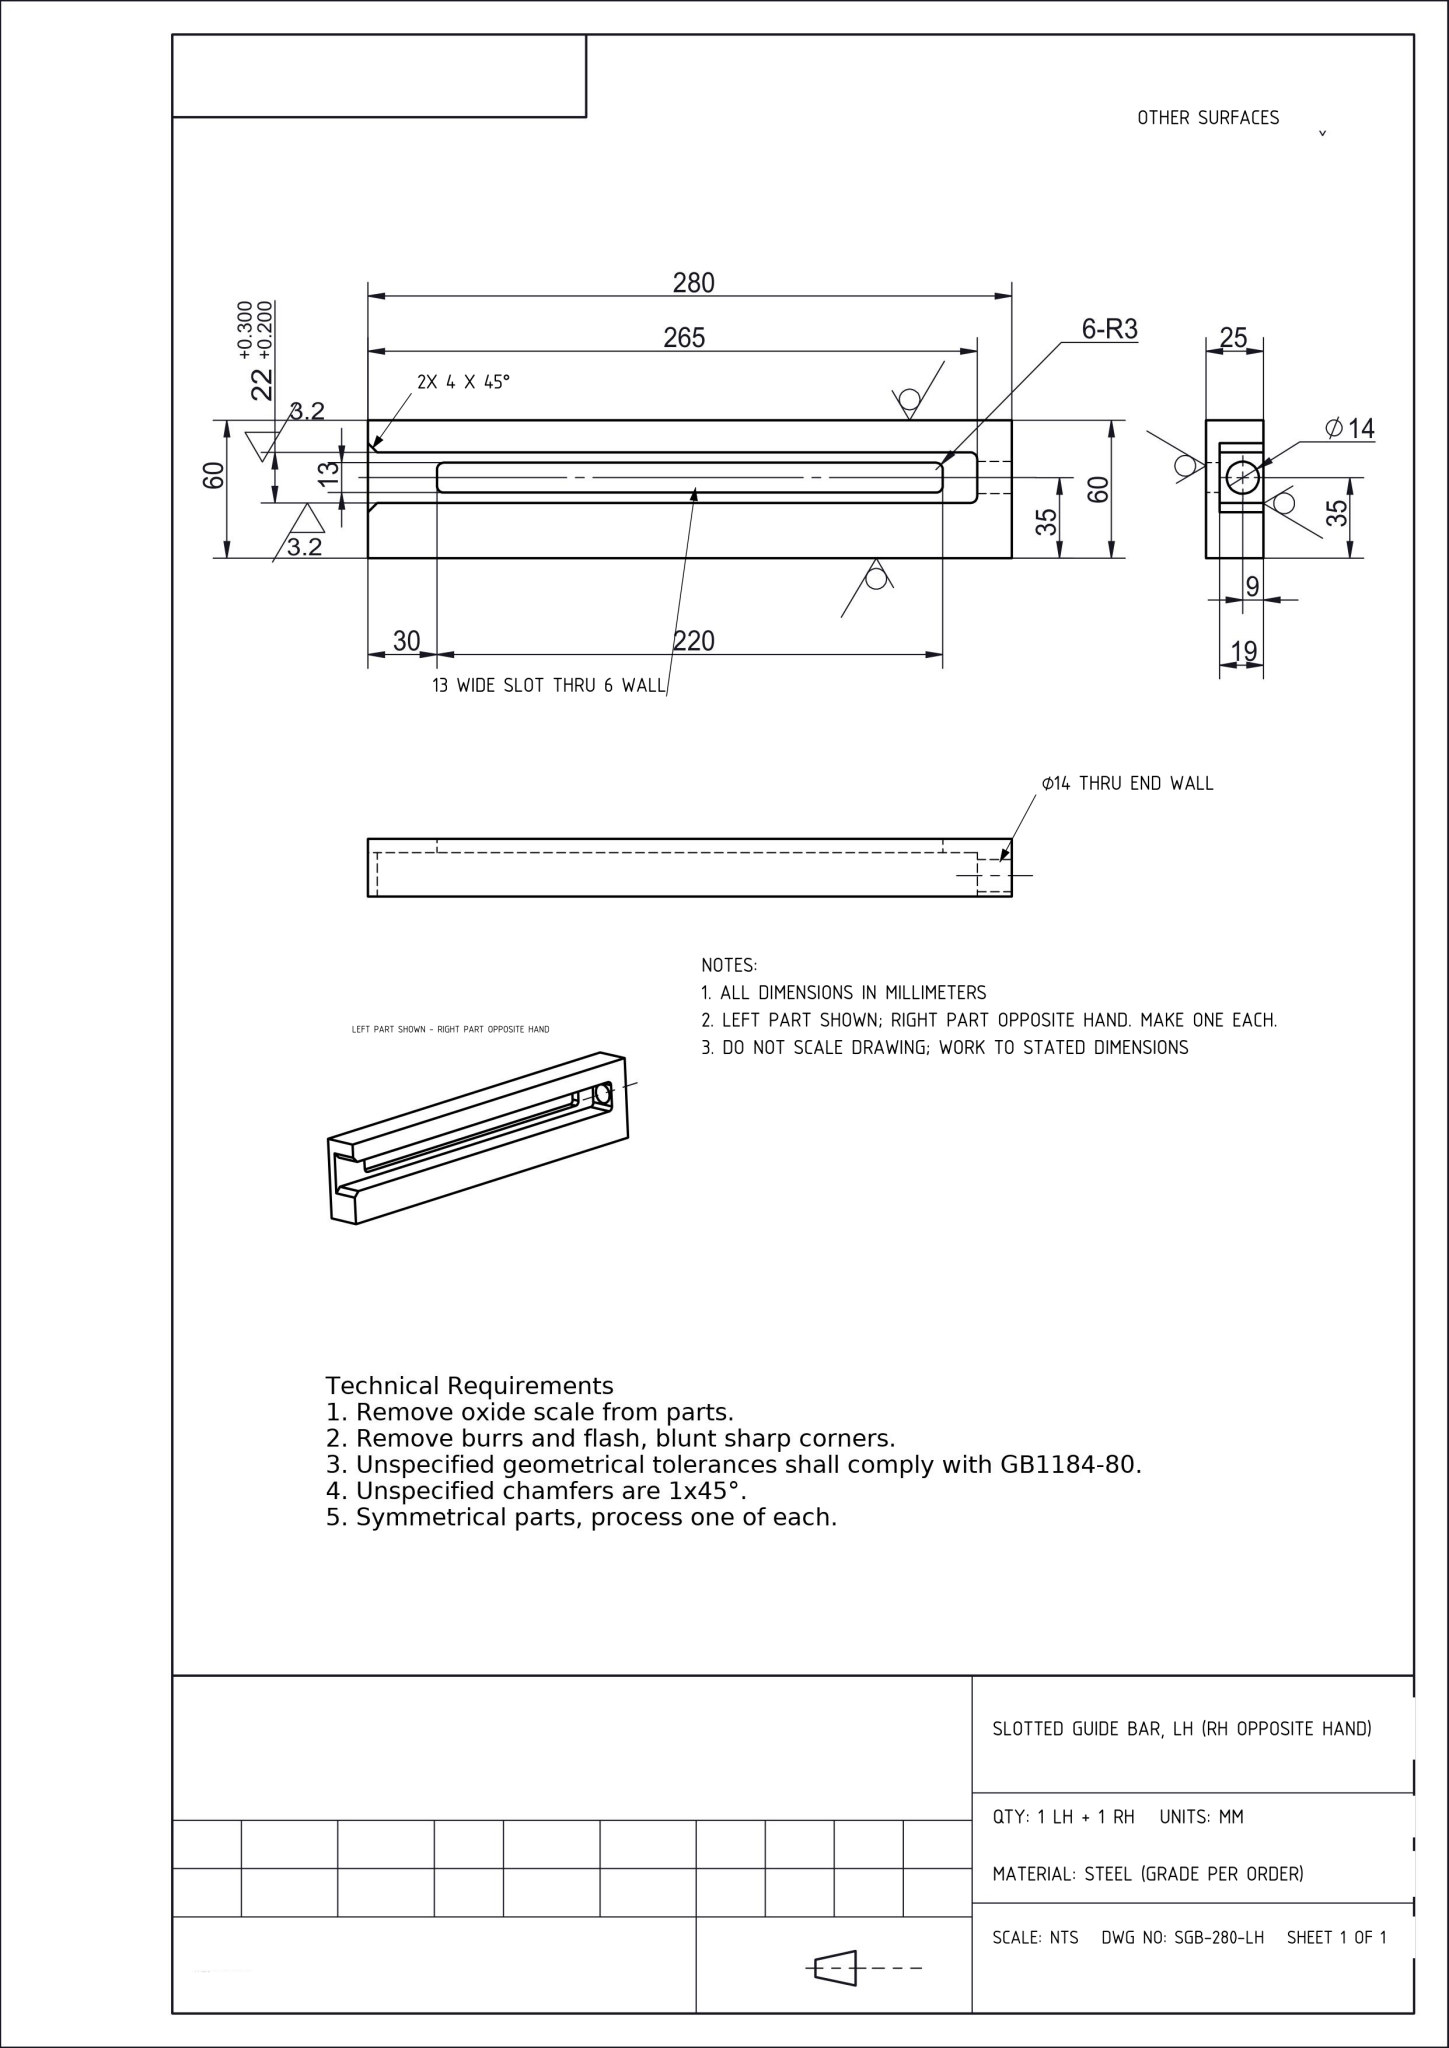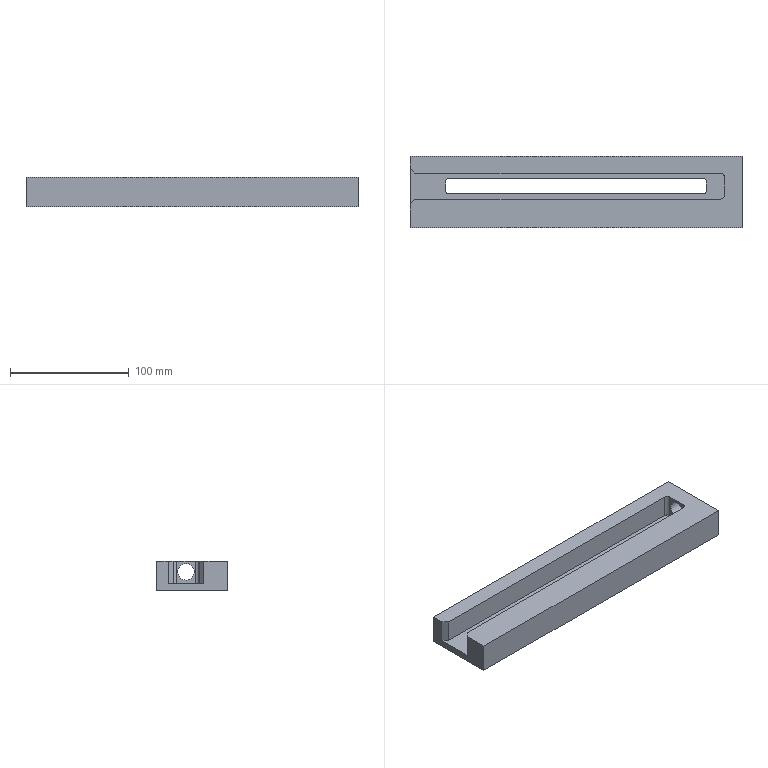Part | NX | mm | 1 solid | 24 faces | box 280 x 60 x 25 mm | volume 289577 mm3 | plane 16 | cylinder 8 | commonest cylinder face diameters 6 x6 14 x2
STEP:
#1=COLOUR_RGB('',1.,1.,1.);
#2=FILL_AREA_STYLE_COLOUR('',#1);
#3=FILL_AREA_STYLE('',(#2));
#4=SURFACE_STYLE_FILL_AREA(#3);
#5=SURFACE_SIDE_STYLE('',(#4));
#6=SURFACE_STYLE_USAGE(.BOTH.,#5);
#7=PRESENTATION_STYLE_ASSIGNMENT((#6));
#8=CARTESIAN_POINT('',(125.,5.,23.));
#9=VERTEX_POINT('',#8);
#10=CARTESIAN_POINT('',(125.,5.,9.));
#11=VERTEX_POINT('',#10);
#12=CARTESIAN_POINT('',(125.,5.,16.));
#13=DIRECTION('',(1.,-0.,-0.));
#14=DIRECTION('',(0.,0.,-1.));
#15=AXIS2_PLACEMENT_3D('',#12,#13,#14);
#16=CIRCLE('',#15,7.);
#17=EDGE_CURVE('',#9,#11,#16,.T.);
#18=ORIENTED_EDGE('',*,*,#17,.F.);
#19=CARTESIAN_POINT('',(140.,5.,23.));
#20=VERTEX_POINT('',#19);
#21=CARTESIAN_POINT('',(140.,5.,23.));
#22=DIRECTION('',(1.,-0.,-0.));
#23=VECTOR('',#22,1000.);
#24=LINE('',#21,#23);
#25=EDGE_CURVE('',#9,#20,#24,.T.);
#26=ORIENTED_EDGE('',*,*,#25,.T.);
#27=CARTESIAN_POINT('',(140.,5.,9.));
#28=VERTEX_POINT('',#27);
#29=CARTESIAN_POINT('',(140.,5.,16.));
#30=DIRECTION('',(1.,-0.,-0.));
#31=DIRECTION('',(0.,0.,-1.));
#32=AXIS2_PLACEMENT_3D('',#29,#30,#31);
#33=CIRCLE('',#32,7.);
#34=EDGE_CURVE('',#20,#28,#33,.T.);
#35=ORIENTED_EDGE('',*,*,#34,.T.);
#36=CARTESIAN_POINT('',(140.,5.,9.));
#37=DIRECTION('',(1.,-0.,-0.));
#38=VECTOR('',#37,1000.);
#39=LINE('',#36,#38);
#40=EDGE_CURVE('',#11,#28,#39,.T.);
#41=ORIENTED_EDGE('',*,*,#40,.F.);
#42=EDGE_LOOP('',(#18,#26,#35,#41));
#43=FACE_OUTER_BOUND('',#42,.T.);
#44=CARTESIAN_POINT('',(140.,5.,16.));
#45=DIRECTION('',(1.,-0.,-0.));
#46=DIRECTION('',(0.,0.,-1.));
#47=AXIS2_PLACEMENT_3D('',#44,#45,#46);
#48=CYLINDRICAL_SURFACE('',#47,7.);
#49=ADVANCED_FACE('',(#43),#48,.F.);
#50=CARTESIAN_POINT('',(140.,5.,16.));
#51=DIRECTION('',(1.,-0.,-0.));
#52=DIRECTION('',(0.,0.,-1.));
#53=AXIS2_PLACEMENT_3D('',#50,#51,#52);
#54=CIRCLE('',#53,7.);
#55=EDGE_CURVE('',#28,#20,#54,.T.);
#56=ORIENTED_EDGE('',*,*,#55,.F.);
#57=ORIENTED_EDGE('',*,*,#34,.F.);
#58=EDGE_LOOP('',(#56,#57));
#59=FACE_BOUND('',#58,.T.);
#60=CARTESIAN_POINT('',(140.,-30.,0.));
#61=VERTEX_POINT('',#60);
#62=CARTESIAN_POINT('',(140.,30.,0.));
#63=VERTEX_POINT('',#62);
#64=CARTESIAN_POINT('',(140.,30.,0.));
#65=DIRECTION('',(-0.,1.,-0.));
#66=VECTOR('',#65,1000.);
#67=LINE('',#64,#66);
#68=EDGE_CURVE('',#61,#63,#67,.T.);
#69=ORIENTED_EDGE('',*,*,#68,.T.);
#70=CARTESIAN_POINT('',(140.,30.,25.));
#71=VERTEX_POINT('',#70);
#72=CARTESIAN_POINT('',(140.,30.,25.));
#73=DIRECTION('',(0.,0.,-1.));
#74=VECTOR('',#73,1000.);
#75=LINE('',#72,#74);
#76=EDGE_CURVE('',#71,#63,#75,.T.);
#77=ORIENTED_EDGE('',*,*,#76,.F.);
#78=CARTESIAN_POINT('',(140.,-30.,25.));
#79=VERTEX_POINT('',#78);
#80=CARTESIAN_POINT('',(140.,30.,25.));
#81=DIRECTION('',(-0.,1.,-0.));
#82=VECTOR('',#81,1000.);
#83=LINE('',#80,#82);
#84=EDGE_CURVE('',#79,#71,#83,.T.);
#85=ORIENTED_EDGE('',*,*,#84,.F.);
#86=CARTESIAN_POINT('',(140.,-30.,25.));
#87=DIRECTION('',(0.,0.,-1.));
#88=VECTOR('',#87,1000.);
#89=LINE('',#86,#88);
#90=EDGE_CURVE('',#79,#61,#89,.T.);
#91=ORIENTED_EDGE('',*,*,#90,.T.);
#92=EDGE_LOOP('',(#69,#77,#85,#91));
#93=FACE_OUTER_BOUND('',#92,.T.);
#94=CARTESIAN_POINT('',(140.,30.,25.));
#95=DIRECTION('',(-1.,0.,-0.));
#96=DIRECTION('',(-0.,-0.,1.));
#97=AXIS2_PLACEMENT_3D('',#94,#95,#96);
#98=PLANE('',#97);
#99=ADVANCED_FACE('',(#59,#93),#98,.F.);
#100=CARTESIAN_POINT('',(-140.,30.,0.));
#101=VERTEX_POINT('',#100);
#102=CARTESIAN_POINT('',(-140.,30.,0.));
#103=DIRECTION('',(-1.,0.,0.));
#104=VECTOR('',#103,1000.);
#105=LINE('',#102,#104);
#106=EDGE_CURVE('',#63,#101,#105,.T.);
#107=ORIENTED_EDGE('',*,*,#106,.T.);
#108=CARTESIAN_POINT('',(-140.,30.,25.));
#109=VERTEX_POINT('',#108);
#110=CARTESIAN_POINT('',(-140.,30.,25.));
#111=DIRECTION('',(0.,0.,-1.));
#112=VECTOR('',#111,1000.);
#113=LINE('',#110,#112);
#114=EDGE_CURVE('',#109,#101,#113,.T.);
#115=ORIENTED_EDGE('',*,*,#114,.F.);
#116=CARTESIAN_POINT('',(-140.,30.,25.));
#117=DIRECTION('',(-1.,0.,0.));
#118=VECTOR('',#117,1000.);
#119=LINE('',#116,#118);
#120=EDGE_CURVE('',#71,#109,#119,.T.);
#121=ORIENTED_EDGE('',*,*,#120,.F.);
#122=ORIENTED_EDGE('',*,*,#76,.T.);
#123=EDGE_LOOP('',(#107,#115,#121,#122));
#124=FACE_OUTER_BOUND('',#123,.T.);
#125=CARTESIAN_POINT('',(-140.,30.,25.));
#126=DIRECTION('',(0.,-1.,-0.));
#127=DIRECTION('',(0.,0.,-1.));
#128=AXIS2_PLACEMENT_3D('',#125,#126,#127);
#129=PLANE('',#128);
#130=ADVANCED_FACE('',(#124),#129,.F.);
#131=CARTESIAN_POINT('',(-140.,-10.,25.));
#132=VERTEX_POINT('',#131);
#133=CARTESIAN_POINT('',(-140.,-30.,25.));
#134=VERTEX_POINT('',#133);
#135=CARTESIAN_POINT('',(-140.,30.,25.));
#136=DIRECTION('',(0.,-1.,0.));
#137=VECTOR('',#136,1000.);
#138=LINE('',#135,#137);
#139=EDGE_CURVE('',#132,#134,#138,.T.);
#140=ORIENTED_EDGE('',*,*,#139,.F.);
#141=CARTESIAN_POINT('',(-140.,-10.,6.));
#142=VERTEX_POINT('',#141);
#143=CARTESIAN_POINT('',(-140.,-10.,25.));
#144=DIRECTION('',(-0.,-0.,-1.));
#145=VECTOR('',#144,1000.);
#146=LINE('',#143,#145);
#147=EDGE_CURVE('',#132,#142,#146,.T.);
#148=ORIENTED_EDGE('',*,*,#147,.T.);
#149=CARTESIAN_POINT('',(-140.,20.,6.));
#150=VERTEX_POINT('',#149);
#151=CARTESIAN_POINT('',(-140.,30.,6.));
#152=DIRECTION('',(0.,-1.,0.));
#153=VECTOR('',#152,1000.);
#154=LINE('',#151,#153);
#155=EDGE_CURVE('',#150,#142,#154,.T.);
#156=ORIENTED_EDGE('',*,*,#155,.F.);
#157=CARTESIAN_POINT('',(-140.,20.,25.));
#158=VERTEX_POINT('',#157);
#159=CARTESIAN_POINT('',(-140.,20.,25.));
#160=DIRECTION('',(0.,0.,1.));
#161=VECTOR('',#160,1000.);
#162=LINE('',#159,#161);
#163=EDGE_CURVE('',#150,#158,#162,.T.);
#164=ORIENTED_EDGE('',*,*,#163,.T.);
#165=CARTESIAN_POINT('',(-140.,30.,25.));
#166=DIRECTION('',(0.,-1.,0.));
#167=VECTOR('',#166,1000.);
#168=LINE('',#165,#167);
#169=EDGE_CURVE('',#109,#158,#168,.T.);
#170=ORIENTED_EDGE('',*,*,#169,.F.);
#171=ORIENTED_EDGE('',*,*,#114,.T.);
#172=CARTESIAN_POINT('',(-140.,-30.,0.));
#173=VERTEX_POINT('',#172);
#174=CARTESIAN_POINT('',(-140.,30.,0.));
#175=DIRECTION('',(0.,-1.,0.));
#176=VECTOR('',#175,1000.);
#177=LINE('',#174,#176);
#178=EDGE_CURVE('',#101,#173,#177,.T.);
#179=ORIENTED_EDGE('',*,*,#178,.T.);
#180=CARTESIAN_POINT('',(-140.,-30.,25.));
#181=DIRECTION('',(0.,0.,-1.));
#182=VECTOR('',#181,1000.);
#183=LINE('',#180,#182);
#184=EDGE_CURVE('',#134,#173,#183,.T.);
#185=ORIENTED_EDGE('',*,*,#184,.F.);
#186=EDGE_LOOP('',(#140,#148,#156,#164,#170,#171,#179,#185));
#187=FACE_OUTER_BOUND('',#186,.T.);
#188=CARTESIAN_POINT('',(-140.,30.,25.));
#189=DIRECTION('',(1.,-0.,0.));
#190=DIRECTION('',(0.,0.,-1.));
#191=AXIS2_PLACEMENT_3D('',#188,#189,#190);
#192=PLANE('',#191);
#193=ADVANCED_FACE('',(#187),#192,.F.);
#194=CARTESIAN_POINT('',(-140.,-30.,0.));
#195=DIRECTION('',(1.,-0.,-0.));
#196=VECTOR('',#195,1000.);
#197=LINE('',#194,#196);
#198=EDGE_CURVE('',#173,#61,#197,.T.);
#199=ORIENTED_EDGE('',*,*,#198,.T.);
#200=ORIENTED_EDGE('',*,*,#90,.F.);
#201=CARTESIAN_POINT('',(-140.,-30.,25.));
#202=DIRECTION('',(1.,-0.,-0.));
#203=VECTOR('',#202,1000.);
#204=LINE('',#201,#203);
#205=EDGE_CURVE('',#134,#79,#204,.T.);
#206=ORIENTED_EDGE('',*,*,#205,.F.);
#207=ORIENTED_EDGE('',*,*,#184,.T.);
#208=EDGE_LOOP('',(#199,#200,#206,#207));
#209=FACE_OUTER_BOUND('',#208,.T.);
#210=CARTESIAN_POINT('',(-140.,-30.,25.));
#211=DIRECTION('',(-0.,1.,0.));
#212=DIRECTION('',(-0.,-0.,1.));
#213=AXIS2_PLACEMENT_3D('',#210,#211,#212);
#214=PLANE('',#213);
#215=ADVANCED_FACE('',(#209),#214,.F.);
#216=CARTESIAN_POINT('',(-136.,-6.,25.));
#217=VERTEX_POINT('',#216);
#218=CARTESIAN_POINT('',(122.,-6.,25.));
#219=VERTEX_POINT('',#218);
#220=CARTESIAN_POINT('',(0.,-6.,25.));
#221=DIRECTION('',(1.,0.,-0.));
#222=VECTOR('',#221,1000.);
#223=LINE('',#220,#222);
#224=EDGE_CURVE('',#217,#219,#223,.T.);
#225=ORIENTED_EDGE('',*,*,#224,.F.);
#226=CARTESIAN_POINT('',(-65.,65.,25.));
#227=DIRECTION('',(-0.7071,-0.7071,-0.));
#228=VECTOR('',#227,1000.);
#229=LINE('',#226,#228);
#230=EDGE_CURVE('',#217,#132,#229,.T.);
#231=ORIENTED_EDGE('',*,*,#230,.T.);
#232=ORIENTED_EDGE('',*,*,#139,.T.);
#233=ORIENTED_EDGE('',*,*,#205,.T.);
#234=ORIENTED_EDGE('',*,*,#84,.T.);
#235=ORIENTED_EDGE('',*,*,#120,.T.);
#236=ORIENTED_EDGE('',*,*,#169,.T.);
#237=CARTESIAN_POINT('',(-136.,16.,25.));
#238=VERTEX_POINT('',#237);
#239=CARTESIAN_POINT('',(-60.,-60.,25.));
#240=DIRECTION('',(0.7071,-0.7071,-0.));
#241=VECTOR('',#240,1000.);
#242=LINE('',#239,#241);
#243=EDGE_CURVE('',#158,#238,#242,.T.);
#244=ORIENTED_EDGE('',*,*,#243,.T.);
#245=CARTESIAN_POINT('',(122.,16.,25.));
#246=VERTEX_POINT('',#245);
#247=CARTESIAN_POINT('',(-284.054,16.,25.));
#248=DIRECTION('',(-1.,0.,0.));
#249=VECTOR('',#248,1000.);
#250=LINE('',#247,#249);
#251=EDGE_CURVE('',#246,#238,#250,.T.);
#252=ORIENTED_EDGE('',*,*,#251,.F.);
#253=CARTESIAN_POINT('',(125.,13.,25.));
#254=VERTEX_POINT('',#253);
#255=CARTESIAN_POINT('',(122.,13.,25.));
#256=DIRECTION('',(0.,0.,-1.));
#257=DIRECTION('',(1.,0.,0.));
#258=AXIS2_PLACEMENT_3D('',#255,#256,#257);
#259=CIRCLE('',#258,3.);
#260=EDGE_CURVE('',#246,#254,#259,.T.);
#261=ORIENTED_EDGE('',*,*,#260,.T.);
#262=CARTESIAN_POINT('',(125.,-3.,25.));
#263=VERTEX_POINT('',#262);
#264=CARTESIAN_POINT('',(125.,16.,25.));
#265=DIRECTION('',(-0.,1.,-0.));
#266=VECTOR('',#265,1000.);
#267=LINE('',#264,#266);
#268=EDGE_CURVE('',#263,#254,#267,.T.);
#269=ORIENTED_EDGE('',*,*,#268,.F.);
#270=CARTESIAN_POINT('',(122.,-3.,25.));
#271=DIRECTION('',(0.,0.,-1.));
#272=DIRECTION('',(1.,0.,0.));
#273=AXIS2_PLACEMENT_3D('',#270,#271,#272);
#274=CIRCLE('',#273,3.);
#275=EDGE_CURVE('',#263,#219,#274,.T.);
#276=ORIENTED_EDGE('',*,*,#275,.T.);
#277=EDGE_LOOP('',(#225,#231,#232,#233,#234,#235,#236,#244,#252,#261,#269,#276));
#278=FACE_OUTER_BOUND('',#277,.T.);
#279=CARTESIAN_POINT('',(0.,0.,25.));
#280=DIRECTION('',(0.,-0.,1.));
#281=DIRECTION('',(1.,-0.,-0.));
#282=AXIS2_PLACEMENT_3D('',#279,#280,#281);
#283=PLANE('',#282);
#284=ADVANCED_FACE('',(#278),#283,.T.);
#285=CARTESIAN_POINT('',(-110.,8.5,0.));
#286=VERTEX_POINT('',#285);
#287=CARTESIAN_POINT('',(-110.,1.5,0.));
#288=VERTEX_POINT('',#287);
#289=CARTESIAN_POINT('',(-110.,0.,0.));
#290=DIRECTION('',(0.,-1.,0.));
#291=VECTOR('',#290,1000.);
#292=LINE('',#289,#291);
#293=EDGE_CURVE('',#286,#288,#292,.T.);
#294=ORIENTED_EDGE('',*,*,#293,.T.);
#295=CARTESIAN_POINT('',(-107.,-1.5,0.));
#296=VERTEX_POINT('',#295);
#297=CARTESIAN_POINT('',(-107.,1.5,0.));
#298=DIRECTION('',(-0.,-0.,1.));
#299=DIRECTION('',(1.,0.,-0.));
#300=AXIS2_PLACEMENT_3D('',#297,#298,#299);
#301=CIRCLE('',#300,3.);
#302=EDGE_CURVE('',#288,#296,#301,.T.);
#303=ORIENTED_EDGE('',*,*,#302,.T.);
#304=CARTESIAN_POINT('',(107.,-1.5,0.));
#305=VERTEX_POINT('',#304);
#306=CARTESIAN_POINT('',(0.,-1.5,0.));
#307=DIRECTION('',(1.,-0.,-0.));
#308=VECTOR('',#307,1000.);
#309=LINE('',#306,#308);
#310=EDGE_CURVE('',#296,#305,#309,.T.);
#311=ORIENTED_EDGE('',*,*,#310,.T.);
#312=CARTESIAN_POINT('',(110.,1.5,0.));
#313=VERTEX_POINT('',#312);
#314=CARTESIAN_POINT('',(107.,1.5,0.));
#315=DIRECTION('',(-0.,-0.,1.));
#316=DIRECTION('',(1.,0.,-0.));
#317=AXIS2_PLACEMENT_3D('',#314,#315,#316);
#318=CIRCLE('',#317,3.);
#319=EDGE_CURVE('',#305,#313,#318,.T.);
#320=ORIENTED_EDGE('',*,*,#319,.T.);
#321=CARTESIAN_POINT('',(110.,8.5,0.));
#322=VERTEX_POINT('',#321);
#323=CARTESIAN_POINT('',(110.,0.,0.));
#324=DIRECTION('',(-0.,1.,-0.));
#325=VECTOR('',#324,1000.);
#326=LINE('',#323,#325);
#327=EDGE_CURVE('',#313,#322,#326,.T.);
#328=ORIENTED_EDGE('',*,*,#327,.T.);
#329=CARTESIAN_POINT('',(107.,11.5,0.));
#330=VERTEX_POINT('',#329);
#331=CARTESIAN_POINT('',(107.,8.5,0.));
#332=DIRECTION('',(-0.,-0.,1.));
#333=DIRECTION('',(1.,0.,-0.));
#334=AXIS2_PLACEMENT_3D('',#331,#332,#333);
#335=CIRCLE('',#334,3.);
#336=EDGE_CURVE('',#322,#330,#335,.T.);
#337=ORIENTED_EDGE('',*,*,#336,.T.);
#338=CARTESIAN_POINT('',(-107.,11.5,0.));
#339=VERTEX_POINT('',#338);
#340=CARTESIAN_POINT('',(0.,11.5,0.));
#341=DIRECTION('',(-1.,0.,0.));
#342=VECTOR('',#341,1000.);
#343=LINE('',#340,#342);
#344=EDGE_CURVE('',#330,#339,#343,.T.);
#345=ORIENTED_EDGE('',*,*,#344,.T.);
#346=CARTESIAN_POINT('',(-107.,8.5,0.));
#347=DIRECTION('',(-0.,-0.,1.));
#348=DIRECTION('',(1.,0.,-0.));
#349=AXIS2_PLACEMENT_3D('',#346,#347,#348);
#350=CIRCLE('',#349,3.);
#351=EDGE_CURVE('',#339,#286,#350,.T.);
#352=ORIENTED_EDGE('',*,*,#351,.T.);
#353=EDGE_LOOP('',(#294,#303,#311,#320,#328,#337,#345,#352));
#354=FACE_BOUND('',#353,.T.);
#355=ORIENTED_EDGE('',*,*,#68,.F.);
#356=ORIENTED_EDGE('',*,*,#198,.F.);
#357=ORIENTED_EDGE('',*,*,#178,.F.);
#358=ORIENTED_EDGE('',*,*,#106,.F.);
#359=EDGE_LOOP('',(#355,#356,#357,#358));
#360=FACE_OUTER_BOUND('',#359,.T.);
#361=CARTESIAN_POINT('',(0.,0.,0.));
#362=DIRECTION('',(0.,-0.,1.));
#363=DIRECTION('',(1.,-0.,-0.));
#364=AXIS2_PLACEMENT_3D('',#361,#362,#363);
#365=PLANE('',#364);
#366=ADVANCED_FACE('',(#354,#360),#365,.F.);
#367=CARTESIAN_POINT('',(110.,1.5,6.));
#368=VERTEX_POINT('',#367);
#369=CARTESIAN_POINT('',(110.,8.5,6.));
#370=VERTEX_POINT('',#369);
#371=CARTESIAN_POINT('',(110.,11.5,6.));
#372=DIRECTION('',(-0.,1.,-0.));
#373=VECTOR('',#372,1000.);
#374=LINE('',#371,#373);
#375=EDGE_CURVE('',#368,#370,#374,.T.);
#376=ORIENTED_EDGE('',*,*,#375,.F.);
#377=CARTESIAN_POINT('',(107.,-1.5,6.));
#378=VERTEX_POINT('',#377);
#379=CARTESIAN_POINT('',(107.,1.5,6.));
#380=DIRECTION('',(0.,0.,-1.));
#381=DIRECTION('',(1.,0.,0.));
#382=AXIS2_PLACEMENT_3D('',#379,#380,#381);
#383=CIRCLE('',#382,3.);
#384=EDGE_CURVE('',#368,#378,#383,.T.);
#385=ORIENTED_EDGE('',*,*,#384,.T.);
#386=CARTESIAN_POINT('',(-107.,-1.5,6.));
#387=VERTEX_POINT('',#386);
#388=CARTESIAN_POINT('',(-110.,-1.5,6.));
#389=DIRECTION('',(1.,-0.,-0.));
#390=VECTOR('',#389,1000.);
#391=LINE('',#388,#390);
#392=EDGE_CURVE('',#387,#378,#391,.T.);
#393=ORIENTED_EDGE('',*,*,#392,.F.);
#394=CARTESIAN_POINT('',(-110.,1.5,6.));
#395=VERTEX_POINT('',#394);
#396=CARTESIAN_POINT('',(-107.,1.5,6.));
#397=DIRECTION('',(0.,0.,-1.));
#398=DIRECTION('',(1.,0.,0.));
#399=AXIS2_PLACEMENT_3D('',#396,#397,#398);
#400=CIRCLE('',#399,3.);
#401=EDGE_CURVE('',#387,#395,#400,.T.);
#402=ORIENTED_EDGE('',*,*,#401,.T.);
#403=CARTESIAN_POINT('',(-110.,8.5,6.));
#404=VERTEX_POINT('',#403);
#405=CARTESIAN_POINT('',(-110.,11.5,6.));
#406=DIRECTION('',(0.,-1.,0.));
#407=VECTOR('',#406,1000.);
#408=LINE('',#405,#407);
#409=EDGE_CURVE('',#404,#395,#408,.T.);
#410=ORIENTED_EDGE('',*,*,#409,.F.);
#411=CARTESIAN_POINT('',(-107.,11.5,6.));
#412=VERTEX_POINT('',#411);
#413=CARTESIAN_POINT('',(-107.,8.5,6.));
#414=DIRECTION('',(0.,0.,-1.));
#415=DIRECTION('',(1.,0.,0.));
#416=AXIS2_PLACEMENT_3D('',#413,#414,#415);
#417=CIRCLE('',#416,3.);
#418=EDGE_CURVE('',#404,#412,#417,.T.);
#419=ORIENTED_EDGE('',*,*,#418,.T.);
#420=CARTESIAN_POINT('',(107.,11.5,6.));
#421=VERTEX_POINT('',#420);
#422=CARTESIAN_POINT('',(-110.,11.5,6.));
#423=DIRECTION('',(-1.,0.,0.));
#424=VECTOR('',#423,1000.);
#425=LINE('',#422,#424);
#426=EDGE_CURVE('',#421,#412,#425,.T.);
#427=ORIENTED_EDGE('',*,*,#426,.F.);
#428=CARTESIAN_POINT('',(107.,8.5,6.));
#429=DIRECTION('',(0.,0.,-1.));
#430=DIRECTION('',(1.,0.,0.));
#431=AXIS2_PLACEMENT_3D('',#428,#429,#430);
#432=CIRCLE('',#431,3.);
#433=EDGE_CURVE('',#421,#370,#432,.T.);
#434=ORIENTED_EDGE('',*,*,#433,.T.);
#435=EDGE_LOOP('',(#376,#385,#393,#402,#410,#419,#427,#434));
#436=FACE_BOUND('',#435,.T.);
#437=ORIENTED_EDGE('',*,*,#155,.T.);
#438=CARTESIAN_POINT('',(-136.,-6.,6.));
#439=VERTEX_POINT('',#438);
#440=CARTESIAN_POINT('',(-140.,-10.,6.));
#441=DIRECTION('',(0.7071,0.7071,0.));
#442=VECTOR('',#441,1000.);
#443=LINE('',#440,#442);
#444=EDGE_CURVE('',#142,#439,#443,.T.);
#445=ORIENTED_EDGE('',*,*,#444,.T.);
#446=CARTESIAN_POINT('',(122.,-6.,6.));
#447=VERTEX_POINT('',#446);
#448=CARTESIAN_POINT('',(-284.054,-6.,6.));
#449=DIRECTION('',(1.,0.,-0.));
#450=VECTOR('',#449,1000.);
#451=LINE('',#448,#450);
#452=EDGE_CURVE('',#439,#447,#451,.T.);
#453=ORIENTED_EDGE('',*,*,#452,.T.);
#454=CARTESIAN_POINT('',(125.,-3.,6.));
#455=VERTEX_POINT('',#454);
#456=CARTESIAN_POINT('',(122.,-3.,6.));
#457=DIRECTION('',(-0.,-0.,1.));
#458=DIRECTION('',(1.,0.,0.));
#459=AXIS2_PLACEMENT_3D('',#456,#457,#458);
#460=CIRCLE('',#459,3.);
#461=EDGE_CURVE('',#447,#455,#460,.T.);
#462=ORIENTED_EDGE('',*,*,#461,.T.);
#463=CARTESIAN_POINT('',(125.,13.,6.));
#464=VERTEX_POINT('',#463);
#465=CARTESIAN_POINT('',(125.,16.,6.));
#466=DIRECTION('',(-0.,1.,-0.));
#467=VECTOR('',#466,1000.);
#468=LINE('',#465,#467);
#469=EDGE_CURVE('',#455,#464,#468,.T.);
#470=ORIENTED_EDGE('',*,*,#469,.T.);
#471=CARTESIAN_POINT('',(122.,16.,6.));
#472=VERTEX_POINT('',#471);
#473=CARTESIAN_POINT('',(122.,13.,6.));
#474=DIRECTION('',(-0.,-0.,1.));
#475=DIRECTION('',(1.,0.,0.));
#476=AXIS2_PLACEMENT_3D('',#473,#474,#475);
#477=CIRCLE('',#476,3.);
#478=EDGE_CURVE('',#464,#472,#477,.T.);
#479=ORIENTED_EDGE('',*,*,#478,.T.);
#480=CARTESIAN_POINT('',(-136.,16.,6.));
#481=VERTEX_POINT('',#480);
#482=CARTESIAN_POINT('',(-284.054,16.,6.));
#483=DIRECTION('',(-1.,0.,0.));
#484=VECTOR('',#483,1000.);
#485=LINE('',#482,#484);
#486=EDGE_CURVE('',#472,#481,#485,.T.);
#487=ORIENTED_EDGE('',*,*,#486,.T.);
#488=CARTESIAN_POINT('',(-140.,20.,6.));
#489=DIRECTION('',(-0.7071,0.7071,0.));
#490=VECTOR('',#489,1000.);
#491=LINE('',#488,#490);
#492=EDGE_CURVE('',#481,#150,#491,.T.);
#493=ORIENTED_EDGE('',*,*,#492,.T.);
#494=EDGE_LOOP('',(#437,#445,#453,#462,#470,#479,#487,#493));
#495=FACE_OUTER_BOUND('',#494,.T.);
#496=CARTESIAN_POINT('',(0.,0.,6.));
#497=DIRECTION('',(0.,-0.,1.));
#498=DIRECTION('',(1.,-0.,-0.));
#499=AXIS2_PLACEMENT_3D('',#496,#497,#498);
#500=PLANE('',#499);
#501=ADVANCED_FACE('',(#436,#495),#500,.T.);
#502=ORIENTED_EDGE('',*,*,#452,.F.);
#503=CARTESIAN_POINT('',(-136.,-6.,6.));
#504=DIRECTION('',(0.,0.,1.));
#505=VECTOR('',#504,1000.);
#506=LINE('',#503,#505);
#507=EDGE_CURVE('',#439,#217,#506,.T.);
#508=ORIENTED_EDGE('',*,*,#507,.T.);
#509=ORIENTED_EDGE('',*,*,#224,.T.);
#510=CARTESIAN_POINT('',(122.,-6.,6.));
#511=DIRECTION('',(0.,0.,-1.));
#512=VECTOR('',#511,1000.);
#513=LINE('',#510,#512);
#514=EDGE_CURVE('',#219,#447,#513,.T.);
#515=ORIENTED_EDGE('',*,*,#514,.T.);
#516=EDGE_LOOP('',(#502,#508,#509,#515));
#517=FACE_OUTER_BOUND('',#516,.T.);
#518=CARTESIAN_POINT('',(-284.054,-6.,6.));
#519=DIRECTION('',(0.,-1.,0.));
#520=DIRECTION('',(1.,0.,-0.));
#521=AXIS2_PLACEMENT_3D('',#518,#519,#520);
#522=PLANE('',#521);
#523=ADVANCED_FACE('',(#517),#522,.F.);
#524=ORIENTED_EDGE('',*,*,#251,.T.);
#525=CARTESIAN_POINT('',(-136.,16.,6.));
#526=DIRECTION('',(-0.,-0.,-1.));
#527=VECTOR('',#526,1000.);
#528=LINE('',#525,#527);
#529=EDGE_CURVE('',#238,#481,#528,.T.);
#530=ORIENTED_EDGE('',*,*,#529,.T.);
#531=ORIENTED_EDGE('',*,*,#486,.F.);
#532=CARTESIAN_POINT('',(122.,16.,25.));
#533=DIRECTION('',(-0.,-0.,1.));
#534=VECTOR('',#533,1000.);
#535=LINE('',#532,#534);
#536=EDGE_CURVE('',#472,#246,#535,.T.);
#537=ORIENTED_EDGE('',*,*,#536,.T.);
#538=EDGE_LOOP('',(#524,#530,#531,#537));
#539=FACE_OUTER_BOUND('',#538,.T.);
#540=CARTESIAN_POINT('',(-284.054,16.,6.));
#541=DIRECTION('',(-0.,1.,0.));
#542=DIRECTION('',(-0.,-0.,1.));
#543=AXIS2_PLACEMENT_3D('',#540,#541,#542);
#544=PLANE('',#543);
#545=ADVANCED_FACE('',(#539),#544,.F.);
#546=CARTESIAN_POINT('',(125.,5.,16.));
#547=DIRECTION('',(1.,-0.,-0.));
#548=DIRECTION('',(0.,0.,-1.));
#549=AXIS2_PLACEMENT_3D('',#546,#547,#548);
#550=CIRCLE('',#549,7.);
#551=EDGE_CURVE('',#11,#9,#550,.T.);
#552=ORIENTED_EDGE('',*,*,#551,.T.);
#553=ORIENTED_EDGE('',*,*,#17,.T.);
#554=EDGE_LOOP('',(#552,#553));
#555=FACE_BOUND('',#554,.T.);
#556=ORIENTED_EDGE('',*,*,#469,.F.);
#557=CARTESIAN_POINT('',(125.,-3.,25.));
#558=DIRECTION('',(-0.,-0.,1.));
#559=VECTOR('',#558,1000.);
#560=LINE('',#557,#559);
#561=EDGE_CURVE('',#455,#263,#560,.T.);
#562=ORIENTED_EDGE('',*,*,#561,.T.);
#563=ORIENTED_EDGE('',*,*,#268,.T.);
#564=CARTESIAN_POINT('',(125.,13.,6.));
#565=DIRECTION('',(0.,0.,-1.));
#566=VECTOR('',#565,1000.);
#567=LINE('',#564,#566);
#568=EDGE_CURVE('',#254,#464,#567,.T.);
#569=ORIENTED_EDGE('',*,*,#568,.T.);
#570=EDGE_LOOP('',(#556,#562,#563,#569));
#571=FACE_OUTER_BOUND('',#570,.T.);
#572=CARTESIAN_POINT('',(125.,16.,6.));
#573=DIRECTION('',(1.,-0.,0.));
#574=DIRECTION('',(0.,0.,-1.));
#575=AXIS2_PLACEMENT_3D('',#572,#573,#574);
#576=PLANE('',#575);
#577=ADVANCED_FACE('',(#555,#571),#576,.F.);
#578=ORIENTED_EDGE('',*,*,#25,.F.);
#579=ORIENTED_EDGE('',*,*,#551,.F.);
#580=ORIENTED_EDGE('',*,*,#40,.T.);
#581=ORIENTED_EDGE('',*,*,#55,.T.);
#582=EDGE_LOOP('',(#578,#579,#580,#581));
#583=FACE_OUTER_BOUND('',#582,.T.);
#584=CARTESIAN_POINT('',(140.,5.,16.));
#585=DIRECTION('',(1.,-0.,-0.));
#586=DIRECTION('',(0.,0.,-1.));
#587=AXIS2_PLACEMENT_3D('',#584,#585,#586);
#588=CYLINDRICAL_SURFACE('',#587,7.);
#589=ADVANCED_FACE('',(#583),#588,.F.);
#590=ORIENTED_EDGE('',*,*,#461,.F.);
#591=ORIENTED_EDGE('',*,*,#514,.F.);
#592=ORIENTED_EDGE('',*,*,#275,.F.);
#593=ORIENTED_EDGE('',*,*,#561,.F.);
#594=EDGE_LOOP('',(#590,#591,#592,#593));
#595=FACE_OUTER_BOUND('',#594,.T.);
#596=CARTESIAN_POINT('',(122.,-3.,6.));
#597=DIRECTION('',(0.,0.,-1.));
#598=DIRECTION('',(-1.,0.,0.));
#599=AXIS2_PLACEMENT_3D('',#596,#597,#598);
#600=CYLINDRICAL_SURFACE('',#599,3.);
#601=ADVANCED_FACE('',(#595),#600,.F.);
#602=ORIENTED_EDGE('',*,*,#478,.F.);
#603=ORIENTED_EDGE('',*,*,#568,.F.);
#604=ORIENTED_EDGE('',*,*,#260,.F.);
#605=ORIENTED_EDGE('',*,*,#536,.F.);
#606=EDGE_LOOP('',(#602,#603,#604,#605));
#607=FACE_OUTER_BOUND('',#606,.T.);
#608=CARTESIAN_POINT('',(122.,13.,6.));
#609=DIRECTION('',(0.,0.,-1.));
#610=DIRECTION('',(-1.,0.,0.));
#611=AXIS2_PLACEMENT_3D('',#608,#609,#610);
#612=CYLINDRICAL_SURFACE('',#611,3.);
#613=ADVANCED_FACE('',(#607),#612,.F.);
#614=ORIENTED_EDGE('',*,*,#327,.F.);
#615=CARTESIAN_POINT('',(110.,1.5,6.));
#616=DIRECTION('',(-0.,-0.,1.));
#617=VECTOR('',#616,1000.);
#618=LINE('',#615,#617);
#619=EDGE_CURVE('',#313,#368,#618,.T.);
#620=ORIENTED_EDGE('',*,*,#619,.T.);
#621=ORIENTED_EDGE('',*,*,#375,.T.);
#622=CARTESIAN_POINT('',(110.,8.5,0.));
#623=DIRECTION('',(0.,0.,-1.));
#624=VECTOR('',#623,1000.);
#625=LINE('',#622,#624);
#626=EDGE_CURVE('',#370,#322,#625,.T.);
#627=ORIENTED_EDGE('',*,*,#626,.T.);
#628=EDGE_LOOP('',(#614,#620,#621,#627));
#629=FACE_OUTER_BOUND('',#628,.T.);
#630=CARTESIAN_POINT('',(110.,11.5,-4.));
#631=DIRECTION('',(1.,-0.,0.));
#632=DIRECTION('',(0.,0.,-1.));
#633=AXIS2_PLACEMENT_3D('',#630,#631,#632);
#634=PLANE('',#633);
#635=ADVANCED_FACE('',(#629),#634,.F.);
#636=ORIENTED_EDGE('',*,*,#392,.T.);
#637=CARTESIAN_POINT('',(107.,-1.5,0.));
#638=DIRECTION('',(0.,0.,-1.));
#639=VECTOR('',#638,1000.);
#640=LINE('',#637,#639);
#641=EDGE_CURVE('',#378,#305,#640,.T.);
#642=ORIENTED_EDGE('',*,*,#641,.T.);
#643=ORIENTED_EDGE('',*,*,#310,.F.);
#644=CARTESIAN_POINT('',(-107.,-1.5,6.));
#645=DIRECTION('',(-0.,-0.,1.));
#646=VECTOR('',#645,1000.);
#647=LINE('',#644,#646);
#648=EDGE_CURVE('',#296,#387,#647,.T.);
#649=ORIENTED_EDGE('',*,*,#648,.T.);
#650=EDGE_LOOP('',(#636,#642,#643,#649));
#651=FACE_OUTER_BOUND('',#650,.T.);
#652=CARTESIAN_POINT('',(-110.,-1.5,-4.));
#653=DIRECTION('',(0.,-1.,-0.));
#654=DIRECTION('',(0.,0.,-1.));
#655=AXIS2_PLACEMENT_3D('',#652,#653,#654);
#656=PLANE('',#655);
#657=ADVANCED_FACE('',(#651),#656,.F.);
#658=ORIENTED_EDGE('',*,*,#409,.T.);
#659=CARTESIAN_POINT('',(-110.,1.5,0.));
#660=DIRECTION('',(0.,0.,-1.));
#661=VECTOR('',#660,1000.);
#662=LINE('',#659,#661);
#663=EDGE_CURVE('',#395,#288,#662,.T.);
#664=ORIENTED_EDGE('',*,*,#663,.T.);
#665=ORIENTED_EDGE('',*,*,#293,.F.);
#666=CARTESIAN_POINT('',(-110.,8.5,6.));
#667=DIRECTION('',(-0.,-0.,1.));
#668=VECTOR('',#667,1000.);
#669=LINE('',#666,#668);
#670=EDGE_CURVE('',#286,#404,#669,.T.);
#671=ORIENTED_EDGE('',*,*,#670,.T.);
#672=EDGE_LOOP('',(#658,#664,#665,#671));
#673=FACE_OUTER_BOUND('',#672,.T.);
#674=CARTESIAN_POINT('',(-110.,11.5,-4.));
#675=DIRECTION('',(-1.,0.,-0.));
#676=DIRECTION('',(-0.,-0.,1.));
#677=AXIS2_PLACEMENT_3D('',#674,#675,#676);
#678=PLANE('',#677);
#679=ADVANCED_FACE('',(#673),#678,.F.);
#680=ORIENTED_EDGE('',*,*,#344,.F.);
#681=CARTESIAN_POINT('',(107.,11.5,6.));
#682=DIRECTION('',(-0.,-0.,1.));
#683=VECTOR('',#682,1000.);
#684=LINE('',#681,#683);
#685=EDGE_CURVE('',#330,#421,#684,.T.);
#686=ORIENTED_EDGE('',*,*,#685,.T.);
#687=ORIENTED_EDGE('',*,*,#426,.T.);
#688=CARTESIAN_POINT('',(-107.,11.5,0.));
#689=DIRECTION('',(0.,0.,-1.));
#690=VECTOR('',#689,1000.);
#691=LINE('',#688,#690);
#692=EDGE_CURVE('',#412,#339,#691,.T.);
#693=ORIENTED_EDGE('',*,*,#692,.T.);
#694=EDGE_LOOP('',(#680,#686,#687,#693));
#695=FACE_OUTER_BOUND('',#694,.T.);
#696=CARTESIAN_POINT('',(-110.,11.5,-4.));
#697=DIRECTION('',(-0.,1.,0.));
#698=DIRECTION('',(-0.,-0.,1.));
#699=AXIS2_PLACEMENT_3D('',#696,#697,#698);
#700=PLANE('',#699);
#701=ADVANCED_FACE('',(#695),#700,.F.);
#702=ORIENTED_EDGE('',*,*,#319,.F.);
#703=ORIENTED_EDGE('',*,*,#641,.F.);
#704=ORIENTED_EDGE('',*,*,#384,.F.);
#705=ORIENTED_EDGE('',*,*,#619,.F.);
#706=EDGE_LOOP('',(#702,#703,#704,#705));
#707=FACE_OUTER_BOUND('',#706,.T.);
#708=CARTESIAN_POINT('',(107.,1.5,-4.));
#709=DIRECTION('',(0.,0.,-1.));
#710=DIRECTION('',(-1.,0.,0.));
#711=AXIS2_PLACEMENT_3D('',#708,#709,#710);
#712=CYLINDRICAL_SURFACE('',#711,3.);
#713=ADVANCED_FACE('',(#707),#712,.F.);
#714=ORIENTED_EDGE('',*,*,#336,.F.);
#715=ORIENTED_EDGE('',*,*,#626,.F.);
#716=ORIENTED_EDGE('',*,*,#433,.F.);
#717=ORIENTED_EDGE('',*,*,#685,.F.);
#718=EDGE_LOOP('',(#714,#715,#716,#717));
#719=FACE_OUTER_BOUND('',#718,.T.);
#720=CARTESIAN_POINT('',(107.,8.5,-4.));
#721=DIRECTION('',(0.,0.,-1.));
#722=DIRECTION('',(-1.,0.,0.));
#723=AXIS2_PLACEMENT_3D('',#720,#721,#722);
#724=CYLINDRICAL_SURFACE('',#723,3.);
#725=ADVANCED_FACE('',(#719),#724,.F.);
#726=ORIENTED_EDGE('',*,*,#302,.F.);
#727=ORIENTED_EDGE('',*,*,#663,.F.);
#728=ORIENTED_EDGE('',*,*,#401,.F.);
#729=ORIENTED_EDGE('',*,*,#648,.F.);
#730=EDGE_LOOP('',(#726,#727,#728,#729));
#731=FACE_OUTER_BOUND('',#730,.T.);
#732=CARTESIAN_POINT('',(-107.,1.5,-4.));
#733=DIRECTION('',(0.,0.,-1.));
#734=DIRECTION('',(-1.,0.,0.));
#735=AXIS2_PLACEMENT_3D('',#732,#733,#734);
#736=CYLINDRICAL_SURFACE('',#735,3.);
#737=ADVANCED_FACE('',(#731),#736,.F.);
#738=ORIENTED_EDGE('',*,*,#351,.F.);
#739=ORIENTED_EDGE('',*,*,#692,.F.);
#740=ORIENTED_EDGE('',*,*,#418,.F.);
#741=ORIENTED_EDGE('',*,*,#670,.F.);
#742=EDGE_LOOP('',(#738,#739,#740,#741));
#743=FACE_OUTER_BOUND('',#742,.T.);
#744=CARTESIAN_POINT('',(-107.,8.5,-4.));
#745=DIRECTION('',(0.,0.,-1.));
#746=DIRECTION('',(-1.,0.,0.));
#747=AXIS2_PLACEMENT_3D('',#744,#745,#746);
#748=CYLINDRICAL_SURFACE('',#747,3.);
#749=ADVANCED_FACE('',(#743),#748,.F.);
#750=ORIENTED_EDGE('',*,*,#230,.F.);
#751=ORIENTED_EDGE('',*,*,#507,.F.);
#752=ORIENTED_EDGE('',*,*,#444,.F.);
#753=ORIENTED_EDGE('',*,*,#147,.F.);
#754=EDGE_LOOP('',(#750,#751,#752,#753));
#755=FACE_OUTER_BOUND('',#754,.T.);
#756=CARTESIAN_POINT('',(-140.,-10.,25.));
#757=DIRECTION('',(0.7071,-0.7071,0.));
#758=DIRECTION('',(-0.,-0.,-1.));
#759=AXIS2_PLACEMENT_3D('',#756,#757,#758);
#760=PLANE('',#759);
#761=ADVANCED_FACE('',(#755),#760,.F.);
#762=ORIENTED_EDGE('',*,*,#492,.F.);
#763=ORIENTED_EDGE('',*,*,#529,.F.);
#764=ORIENTED_EDGE('',*,*,#243,.F.);
#765=ORIENTED_EDGE('',*,*,#163,.F.);
#766=EDGE_LOOP('',(#762,#763,#764,#765));
#767=FACE_OUTER_BOUND('',#766,.T.);
#768=CARTESIAN_POINT('',(-140.,20.,25.));
#769=DIRECTION('',(0.7071,0.7071,-0.));
#770=DIRECTION('',(0.,0.,1.));
#771=AXIS2_PLACEMENT_3D('',#768,#769,#770);
#772=PLANE('',#771);
#773=ADVANCED_FACE('',(#767),#772,.F.);
#774=CLOSED_SHELL('',(#49,#99,#130,#193,#215,#284,#366,#501,#523,#545,#577,#589,#601,#613,#635,#657,#679,#701,#713,#725,#737,#749,#761,#773));
#775=MANIFOLD_SOLID_BREP('',#774);
#776=CARTESIAN_POINT('',(0.,0.,0.));
#777=DIRECTION('',(0.,0.,1.));
#778=DIRECTION('',(1.,0.,0.));
#779=AXIS2_PLACEMENT_3D('',#776,#777,#778);
#780=(LENGTH_UNIT()NAMED_UNIT(*)SI_UNIT(.MILLI.,.METRE.));
#781=UNCERTAINTY_MEASURE_WITH_UNIT(LENGTH_MEASURE(0.00001),#780,'','');
#782=(NAMED_UNIT(*)PLANE_ANGLE_UNIT()SI_UNIT($,.RADIAN.));
#783=(NAMED_UNIT(*)SI_UNIT($,.STERADIAN.)SOLID_ANGLE_UNIT());
#784=(GEOMETRIC_REPRESENTATION_CONTEXT(3)GLOBAL_UNCERTAINTY_ASSIGNED_CONTEXT((#781))GLOBAL_UNIT_ASSIGNED_CONTEXT((#780,#782,#783))REPRESENTATION_CONTEXT('',''));
#785=ADVANCED_BREP_SHAPE_REPRESENTATION('',(#775,#779),#784);
#786=STYLED_ITEM('',(#7),#785);
#787=(LENGTH_UNIT()NAMED_UNIT(*)SI_UNIT(.MILLI.,.METRE.));
#788=UNCERTAINTY_MEASURE_WITH_UNIT(LENGTH_MEASURE(0.00001),#787,'','');
#789=(NAMED_UNIT(*)PLANE_ANGLE_UNIT()SI_UNIT($,.RADIAN.));
#790=(NAMED_UNIT(*)SI_UNIT($,.STERADIAN.)SOLID_ANGLE_UNIT());
#791=(GEOMETRIC_REPRESENTATION_CONTEXT(3)GLOBAL_UNCERTAINTY_ASSIGNED_CONTEXT((#788))GLOBAL_UNIT_ASSIGNED_CONTEXT((#787,#789,#790))REPRESENTATION_CONTEXT('',''));
#792=MECHANICAL_DESIGN_GEOMETRIC_PRESENTATION_REPRESENTATION('',(#786),#791);
#793=COLOUR_RGB('',1.,1.,1.);
#794=FILL_AREA_STYLE_COLOUR('',#793);
#795=FILL_AREA_STYLE('',(#794));
#796=SURFACE_STYLE_FILL_AREA(#795);
#797=SURFACE_SIDE_STYLE('',(#796));
#798=SURFACE_STYLE_USAGE(.BOTH.,#797);
#799=PRESENTATION_STYLE_ASSIGNMENT((#798));
#800=STYLED_ITEM('',(#799),#775);
#801=(LENGTH_UNIT()NAMED_UNIT(*)SI_UNIT(.MILLI.,.METRE.));
#802=UNCERTAINTY_MEASURE_WITH_UNIT(LENGTH_MEASURE(0.00001),#801,'','');
#803=(NAMED_UNIT(*)PLANE_ANGLE_UNIT()SI_UNIT($,.RADIAN.));
#804=(NAMED_UNIT(*)SI_UNIT($,.STERADIAN.)SOLID_ANGLE_UNIT());
#805=(GEOMETRIC_REPRESENTATION_CONTEXT(3)GLOBAL_UNCERTAINTY_ASSIGNED_CONTEXT((#802))GLOBAL_UNIT_ASSIGNED_CONTEXT((#801,#803,#804))REPRESENTATION_CONTEXT('',''));
#806=MECHANICAL_DESIGN_GEOMETRIC_PRESENTATION_REPRESENTATION('',(#800),#805);
#807=PRESENTATION_LAYER_ASSIGNMENT('','',(#786));
#808=PRESENTATION_LAYER_ASSIGNMENT('','',(#800));